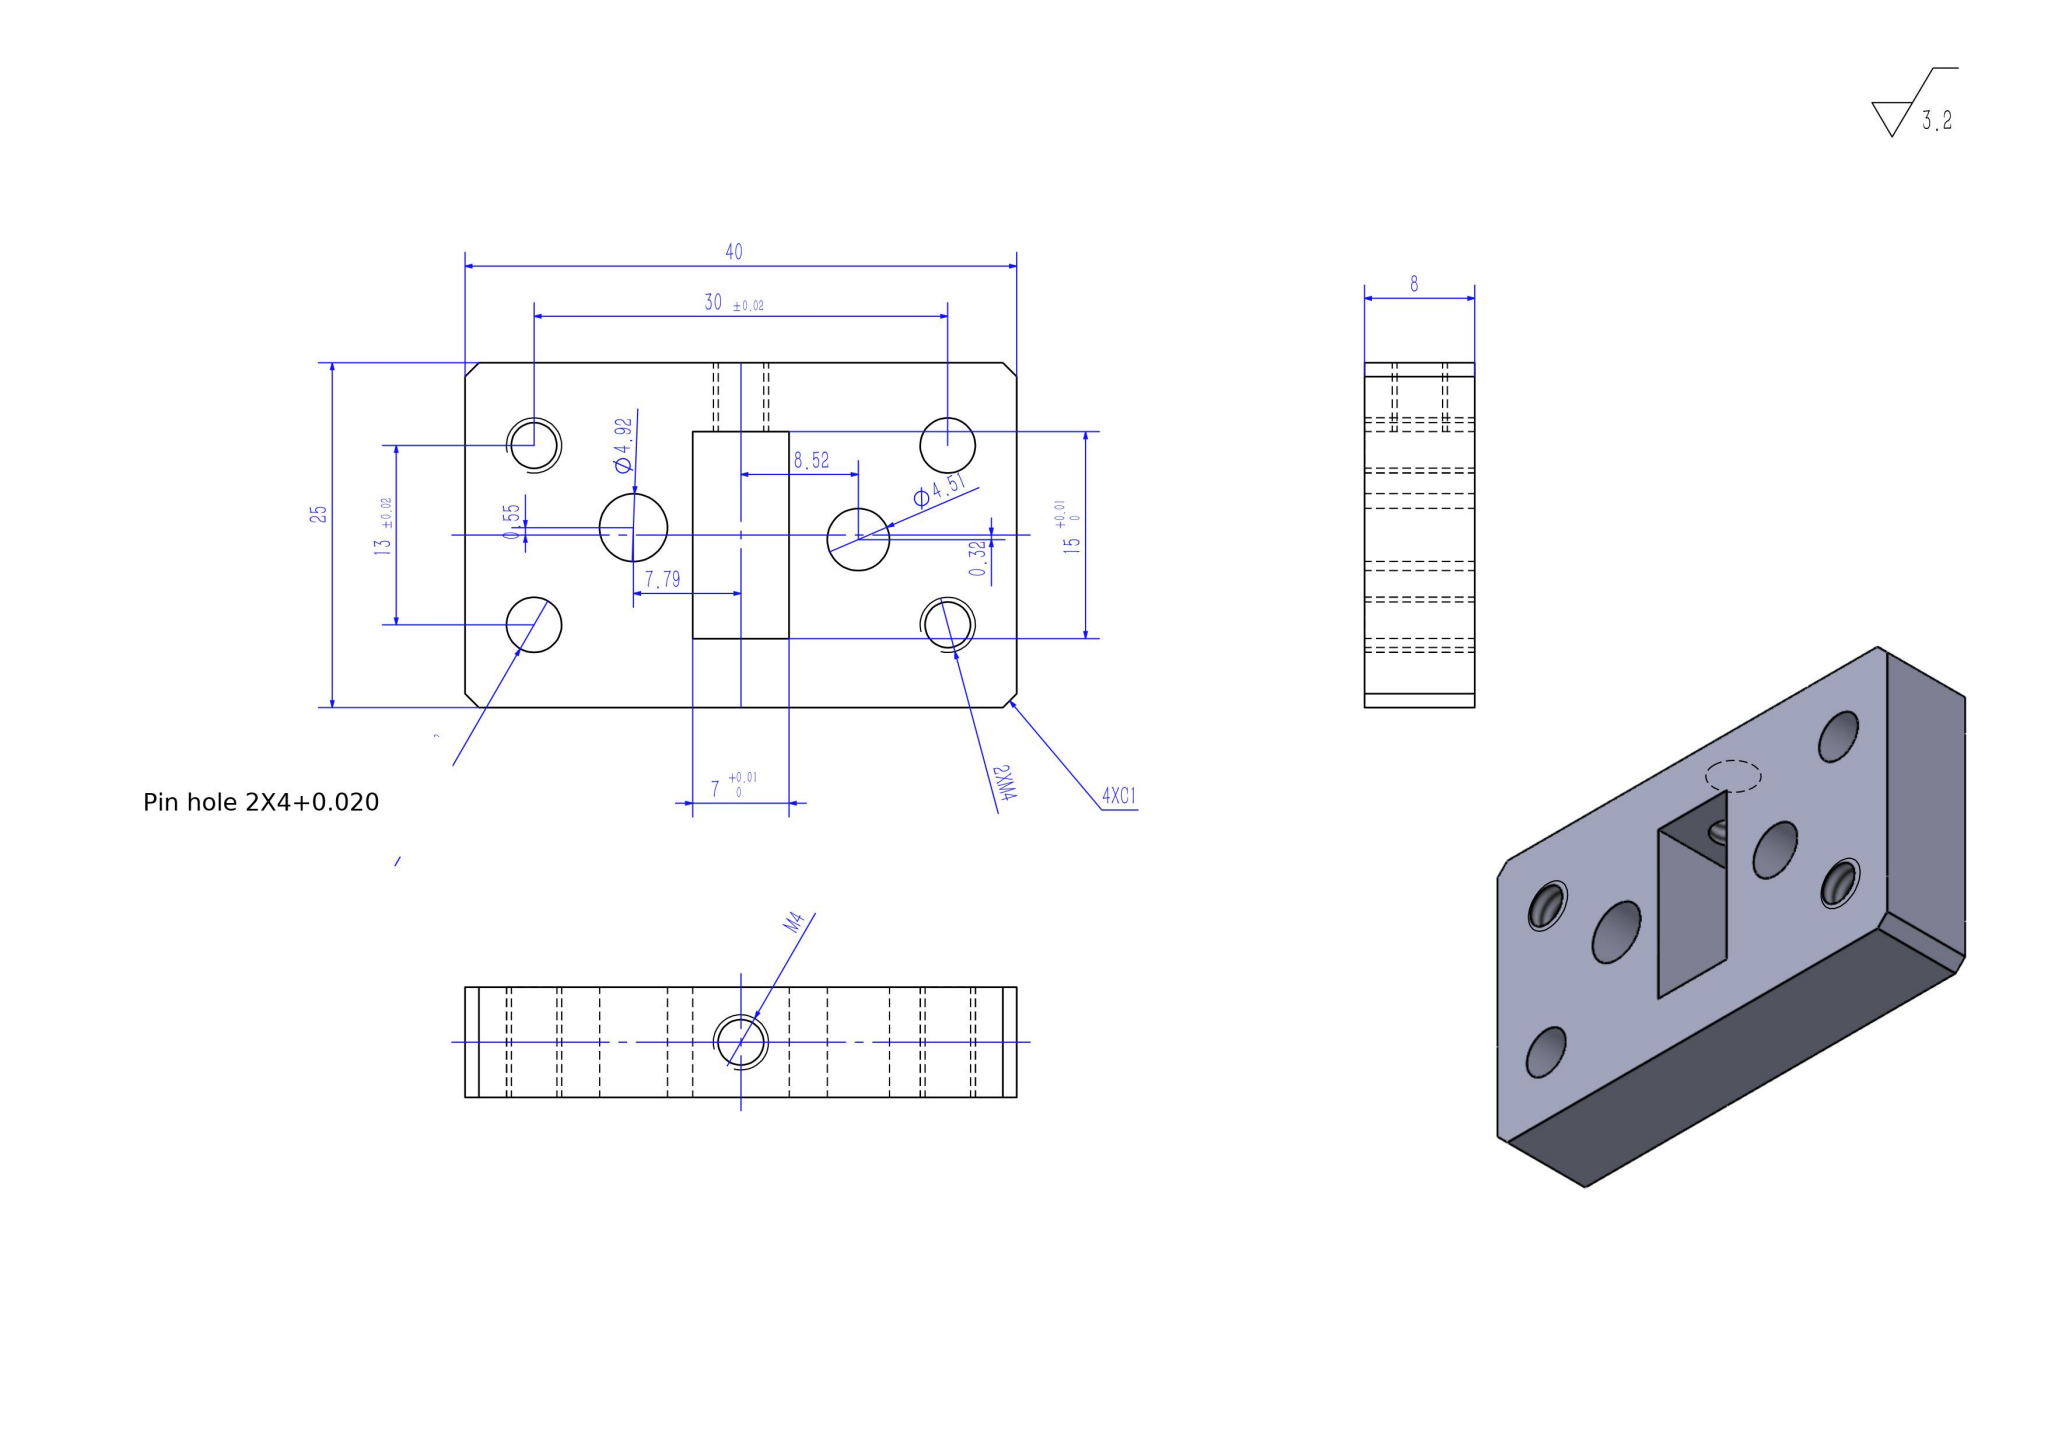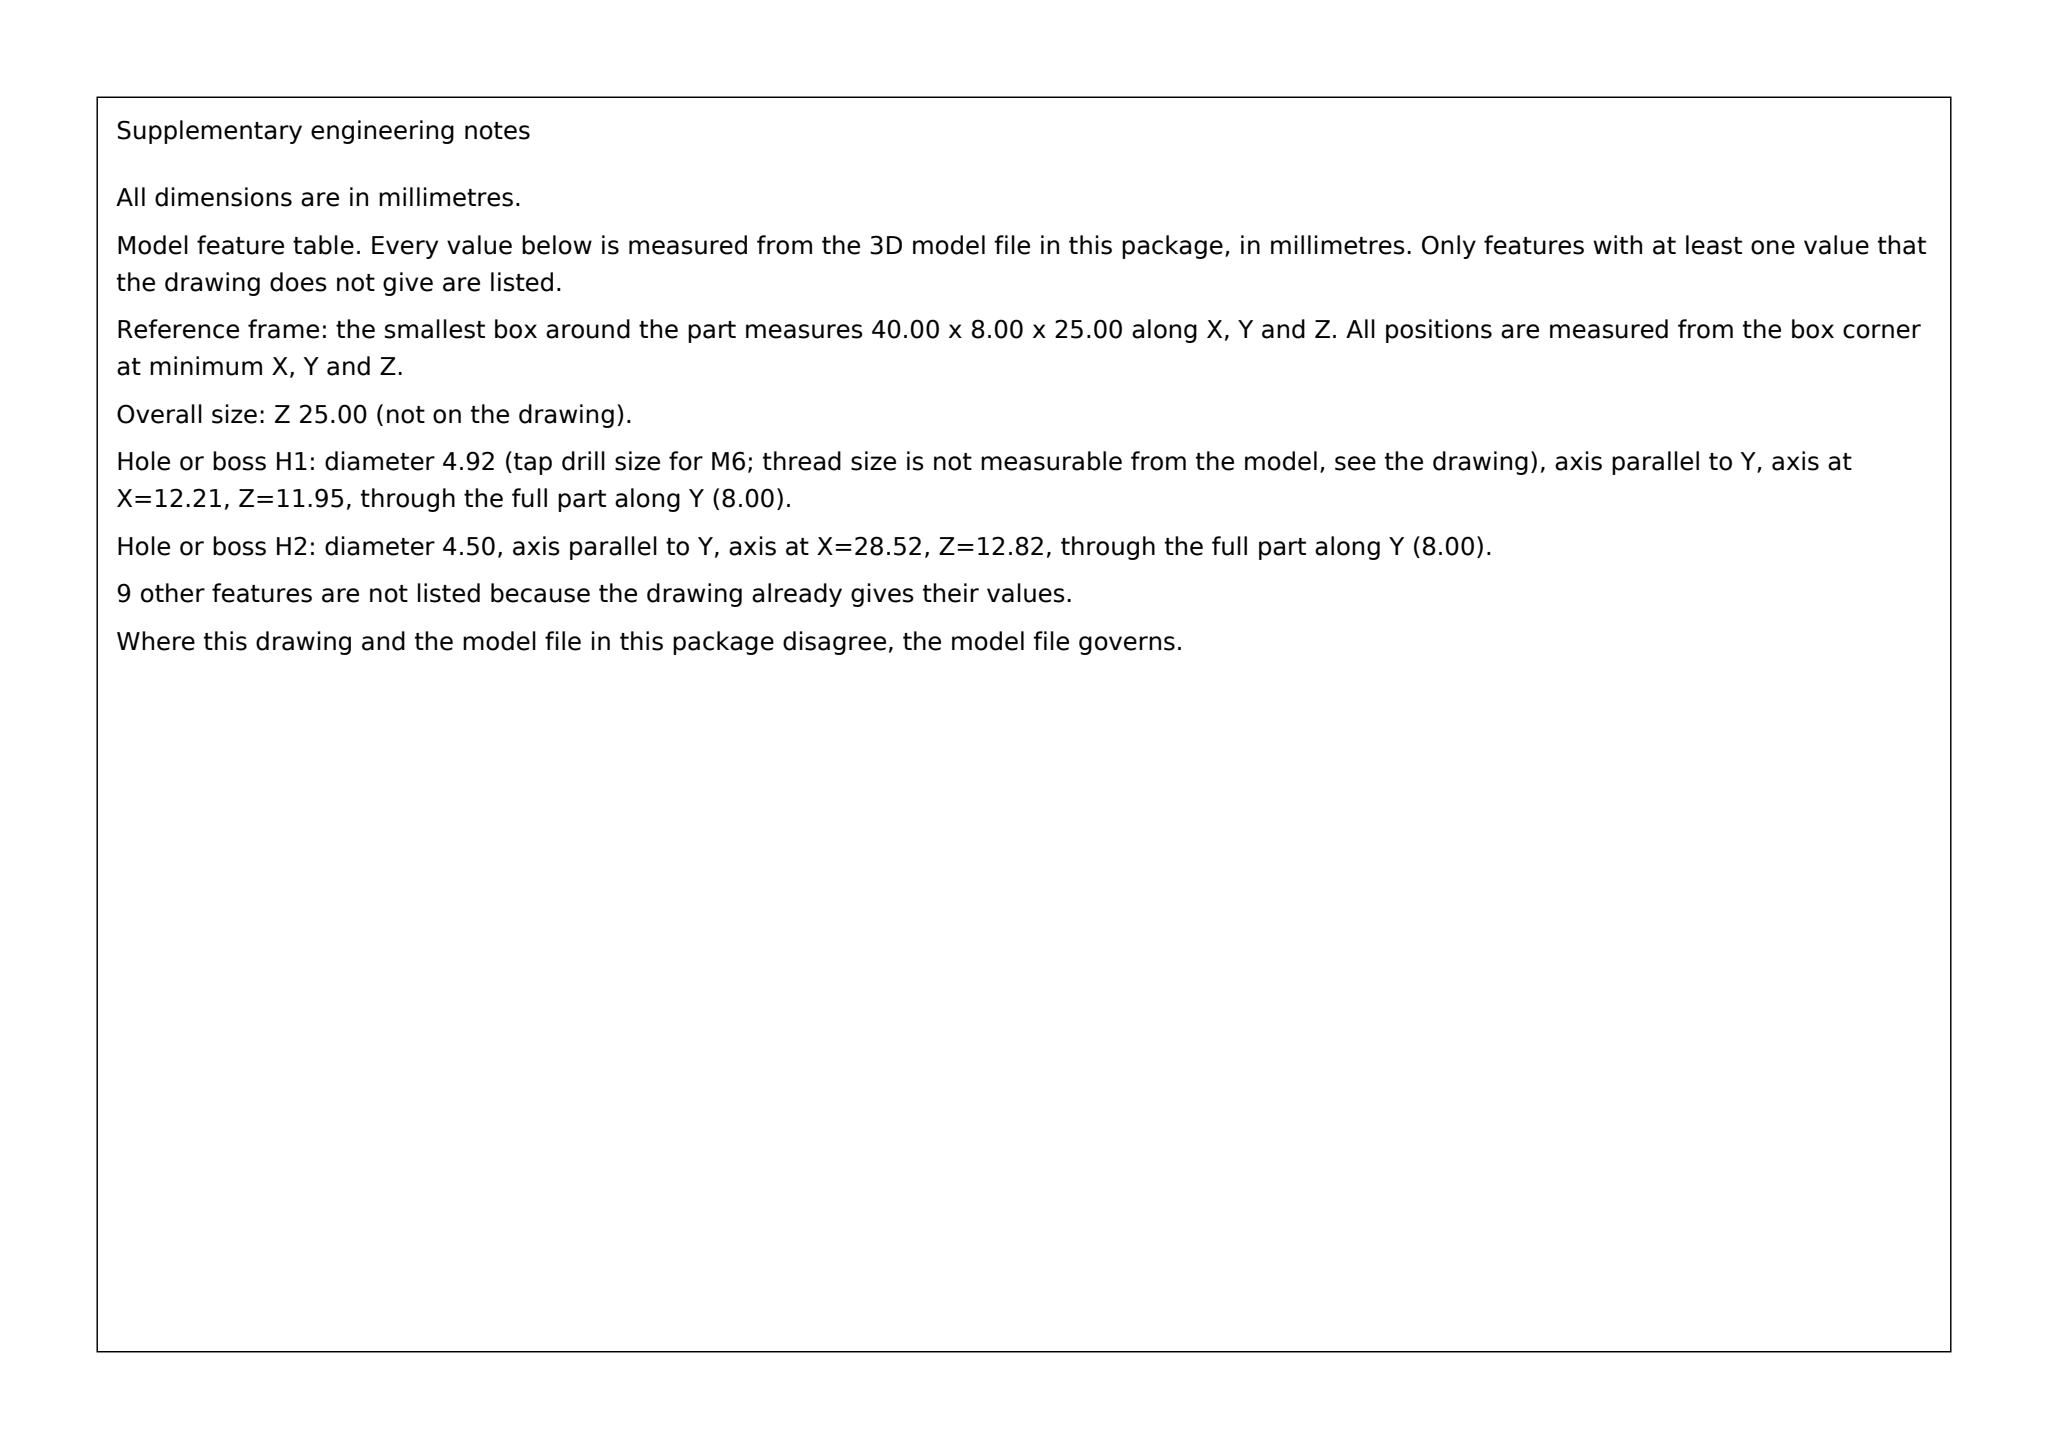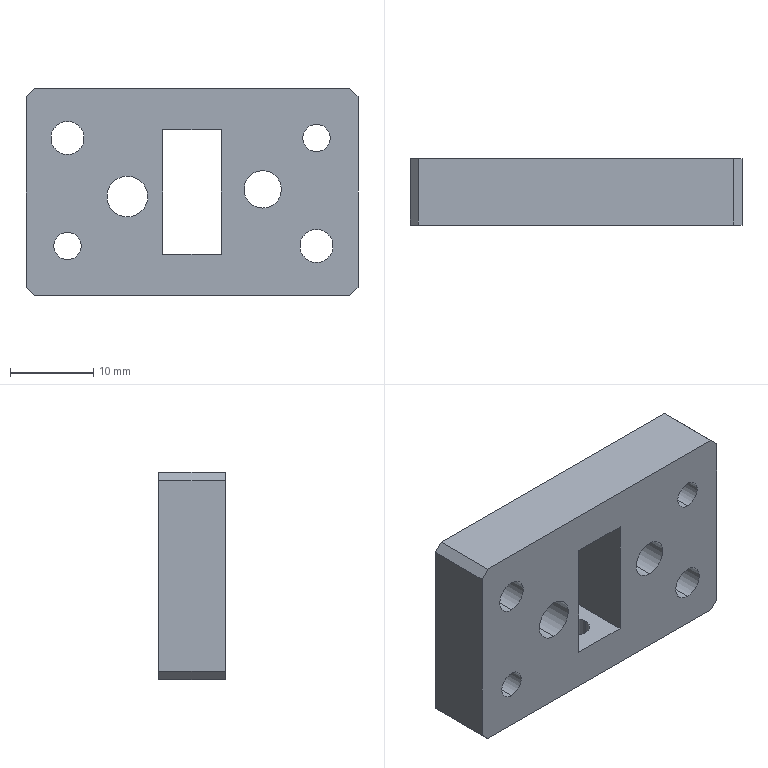Part | SolidWorks | mm | 1 solid | 28 faces | box 40 x 8 x 25 mm | volume 6484 mm3 | cylinder 14 | plane 14 | commonest cylinder face diameters 3.3 x6 4 x4 4.919 x2 4.507 x2
build123d program:
from build123d import *

# Parameters (mm, degrees)
SKETCH1_W             = 40
SKETCH1_H             = 25
BOSS_EXTRUDE1_DEPTH   = 8
SKETCH2_W             = 7
SKETCH2_H             = 15
CUT_EXTRUDE1_DEPTH    = 26
SKETCH3_R             = 2
CUT_EXTRUDE2_DEPTH    = 26
M4_TAPPED_HOLE1_D     = 3.3
M4_TAPPED_HOLE1_DEPTH = 15
M4_TAPPED_HOLE1_TIP   = 0.9914
M4_TAPPED_HOLE2_D     = 3.3
M4_TAPPED_HOLE2_DEPTH = 15
M4_TAPPED_HOLE2_TIP   = 0.9914
CHAMFER1_SIZE         = 1
SKETCH10_R            = 2.459
SKETCH10_R_2          = 2.253
CUT_EXTRUDE3_DEPTH    = 80


with BuildPart() as part:
    # Sketch1 → Boss-Extrude1 (new body)
    with BuildSketch(Plane(origin=(0, 0, 0), x_dir=(1, 0, 0), z_dir=(0, 1, 0))):
        Rectangle(SKETCH1_W, SKETCH1_H)
    extrude(amount=BOSS_EXTRUDE1_DEPTH)

    # Sketch2 → Cut-Extrude1 (cut)
    with BuildSketch(Plane(origin=(0, 8, 0), x_dir=(1, 0, 0), z_dir=(0, 1, 0))):
        Rectangle(SKETCH2_W, SKETCH2_H)
    extrude(amount=-CUT_EXTRUDE1_DEPTH, mode=Mode.SUBTRACT)

    # Sketch3 → Cut-Extrude2 (cut)
    with BuildSketch(Plane(origin=(0, 8, 0), x_dir=(1, 0, 0), z_dir=(0, 1, 0))):
        with Locations(Location((15, 6.5, 0), (0, 0, 270))):
            Circle(SKETCH3_R)
        with Locations(Location((-15, -6.5, 0), (0, 0, 270))):
            Circle(SKETCH3_R)
    extrude(amount=-CUT_EXTRUDE2_DEPTH, mode=Mode.SUBTRACT)

    # M4 Tapped Hole1
    with Locations(Plane(origin=(0, 8, 0), x_dir=(1, 0, 0), z_dir=(0, 1, 0))):
        with Locations((15, -6.5), (-15, 6.5)):
            Hole(M4_TAPPED_HOLE1_D / 2, depth=M4_TAPPED_HOLE1_DEPTH)
            with Locations((0, 0, -(M4_TAPPED_HOLE1_DEPTH + M4_TAPPED_HOLE1_TIP / 2))):  # 118° drill point
                Cone(0, M4_TAPPED_HOLE1_D / 2, M4_TAPPED_HOLE1_TIP, mode=Mode.SUBTRACT)

    # M4 Tapped Hole2
    with Locations(Plane(origin=(0, 0, -12.5), x_dir=(-1, 0, 0), z_dir=(0, 0, -1))):
        with Locations((0, 4)):
            Hole(M4_TAPPED_HOLE2_D / 2, depth=M4_TAPPED_HOLE2_DEPTH)
            with Locations((0, 0, -(M4_TAPPED_HOLE2_DEPTH + M4_TAPPED_HOLE2_TIP / 2))):  # 118° drill point
                Cone(0, M4_TAPPED_HOLE2_D / 2, M4_TAPPED_HOLE2_TIP, mode=Mode.SUBTRACT)

    # Chamfer1
    chamfer1_edges = [part.edges().sort_by_distance(p)[0] for p in [
        (20, 4, 12.5),
        (-20, 4, 12.5),
        (-20, 4, -12.5),
        (20, 4, -12.5),
    ]]
    chamfer(chamfer1_edges, length=CHAMFER1_SIZE)

    # Sketch10 → Cut-Extrude3 (cut)
    with BuildSketch(Plane(origin=(0, 8, 0), x_dir=(1, 0, 0), z_dir=(0, 1, 0))):
        with Locations(Location((-7.788, 0.5465, 0), (0, 0, 270))):
            Circle(SKETCH10_R)
        with Locations(Location((8.516, -0.3188, 0), (0, 0, 270))):
            Circle(SKETCH10_R_2)
    extrude(amount=-CUT_EXTRUDE3_DEPTH, mode=Mode.SUBTRACT)


solid = part.part